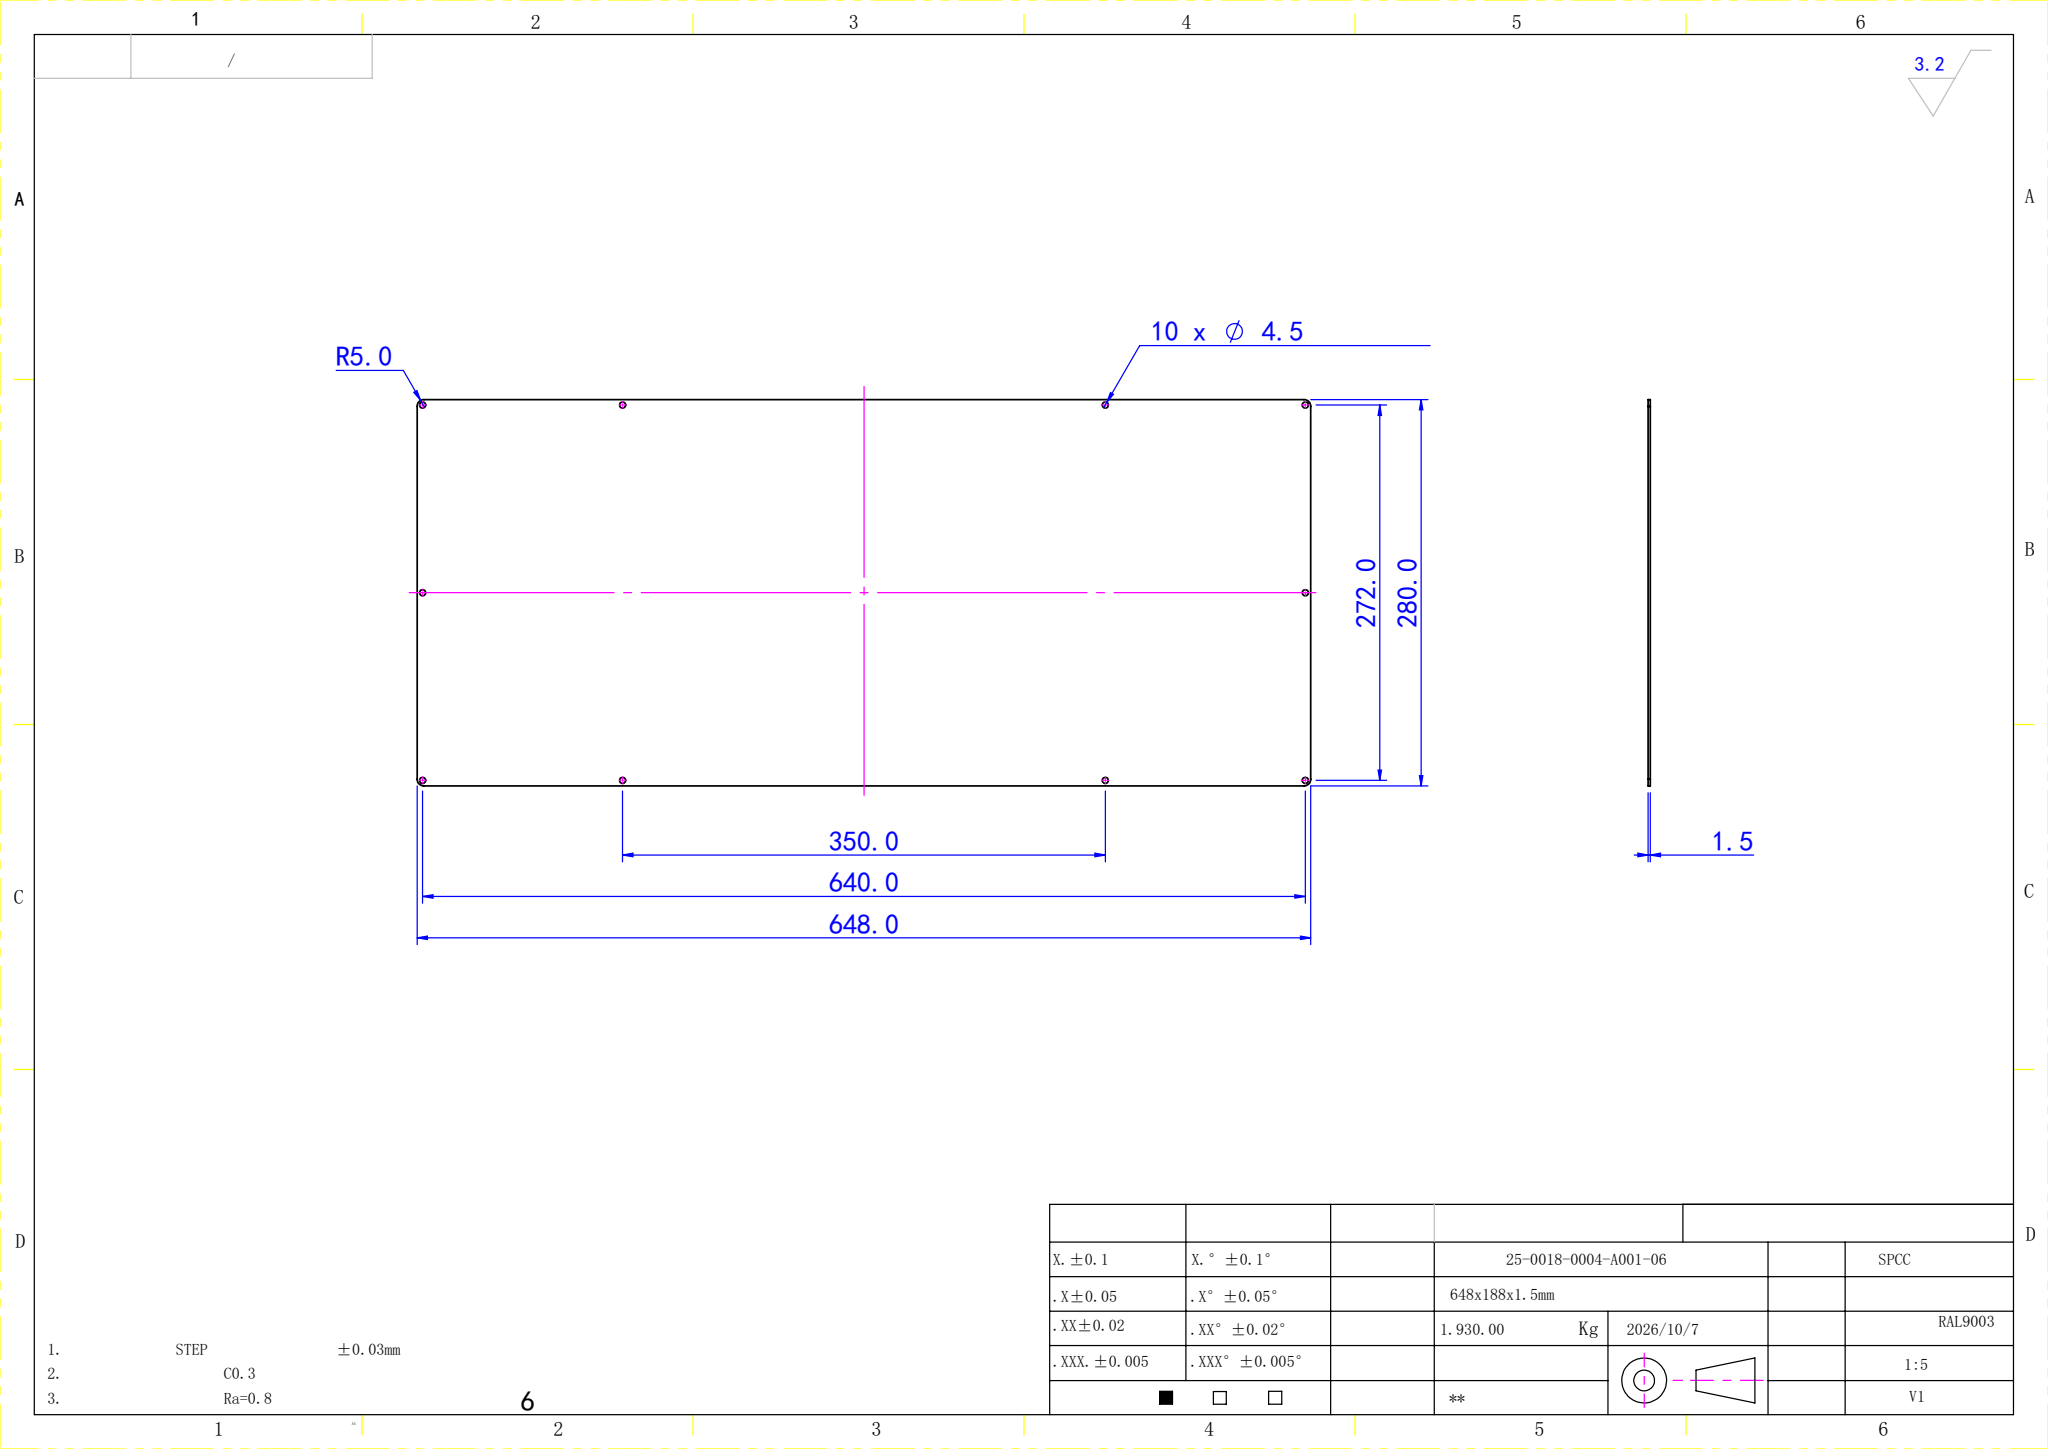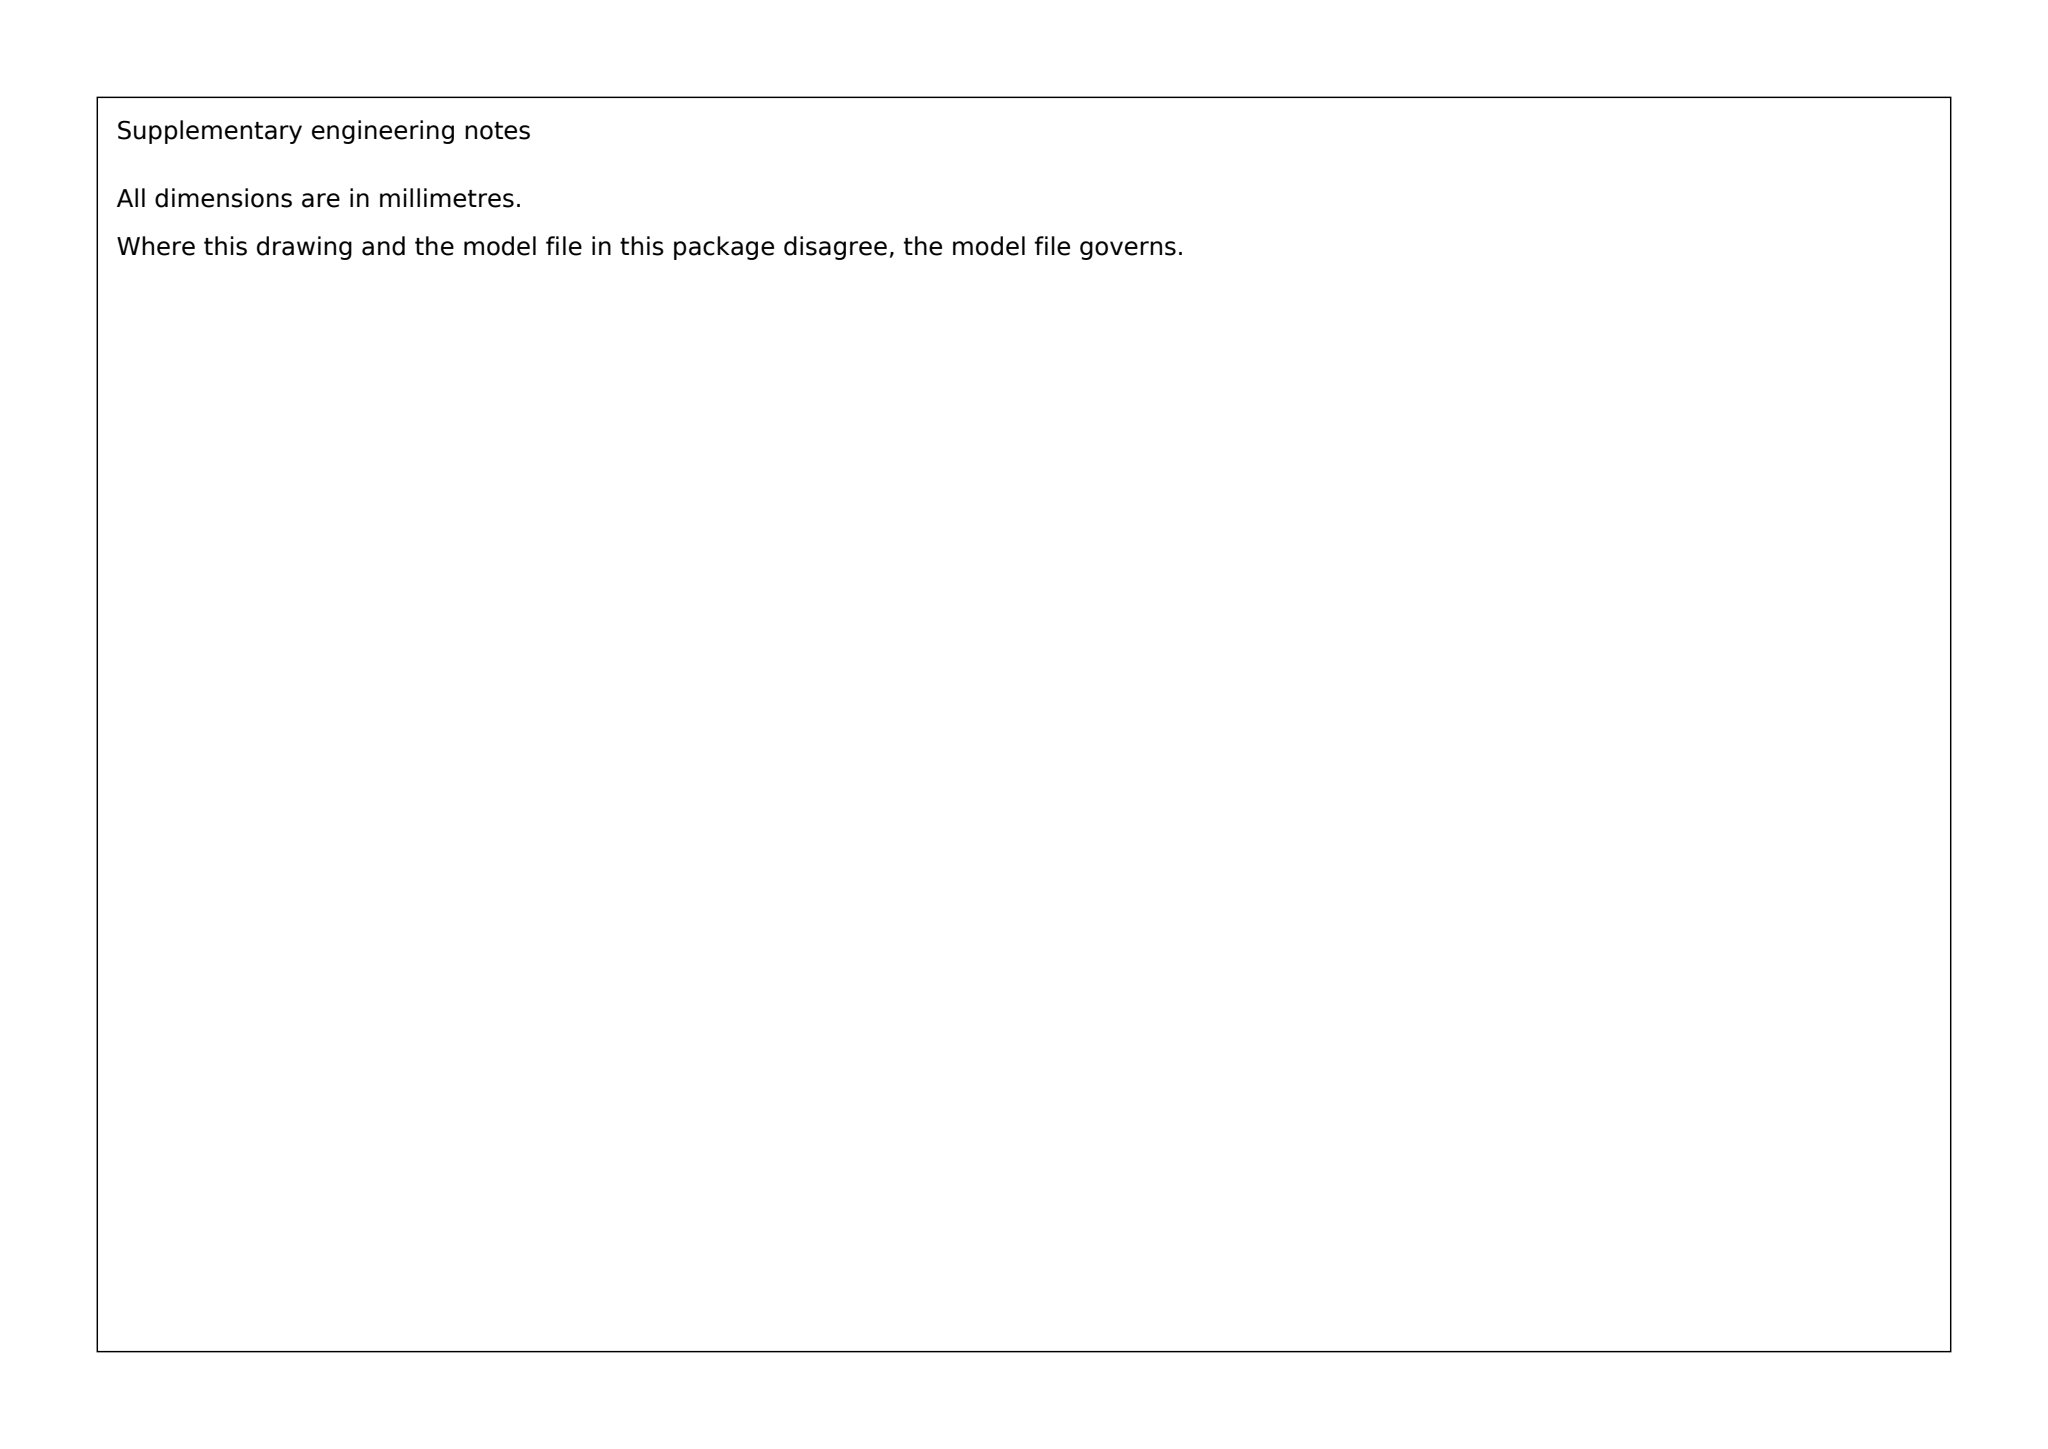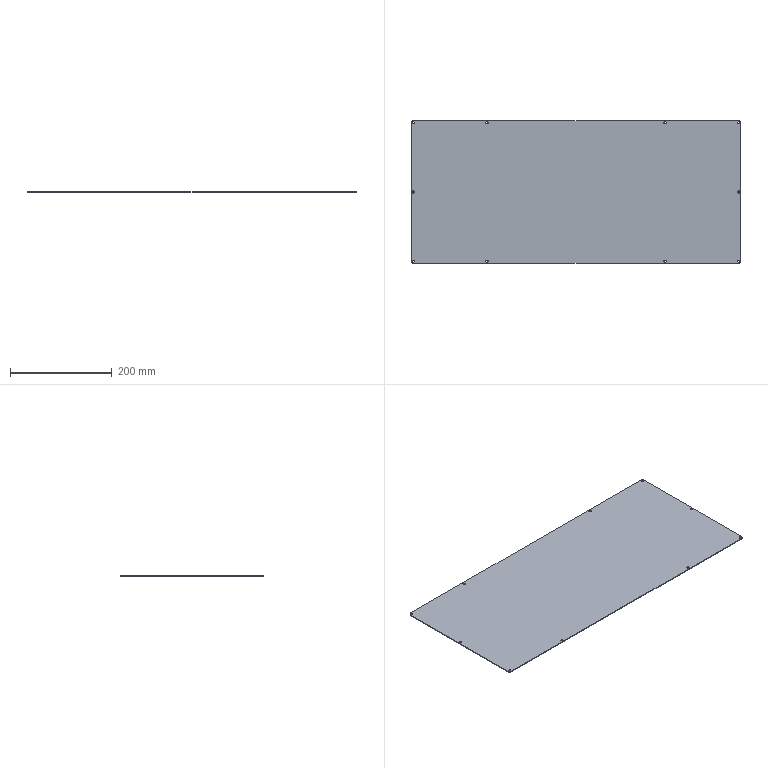Part | SolidWorks | mm | 1 solid | 30 faces | box 648 x 280 x 1.5 mm | volume 271889 mm3 | cylinder 24 | plane 6 | commonest cylinder face diameters 4.5 x20 10 x4
build123d program:
from build123d import *

# Parameters (mm, degrees)
SKETCH1_W            = 648
SKETCH1_H            = 280
BOSS_EXTRUDE1_DEPTH  = 1.5
M4_CLEARANCE_HOLE1_D = 4.5
FILLET1_R            = 5


with BuildPart() as part:
    # Sketch1 → Boss-Extrude1 (new body)
    with BuildSketch(Plane.XY):
        Rectangle(SKETCH1_W, SKETCH1_H)
    extrude(amount=BOSS_EXTRUDE1_DEPTH)

    # M4 Clearance Hole1 (through all)
    with Locations(Plane.XY.offset(1.5)):
        with Locations((-175, 136), (175, 136), (175, -136), (-175, -136), (320, 0), (-320, 0), (-320, 136), (-320, -136), (320, -136), (320, 136)):
            Hole(M4_CLEARANCE_HOLE1_D / 2)

    # Fillet1
    fillet1_edges = [part.edges().sort_by_distance(p)[0] for p in [
        (-324, 140, 0.75),
        (324, 140, 0.75),
        (324, -140, 0.75),
        (-324, -140, 0.75),
    ]]
    fillet(fillet1_edges, radius=FILLET1_R)


solid = part.part